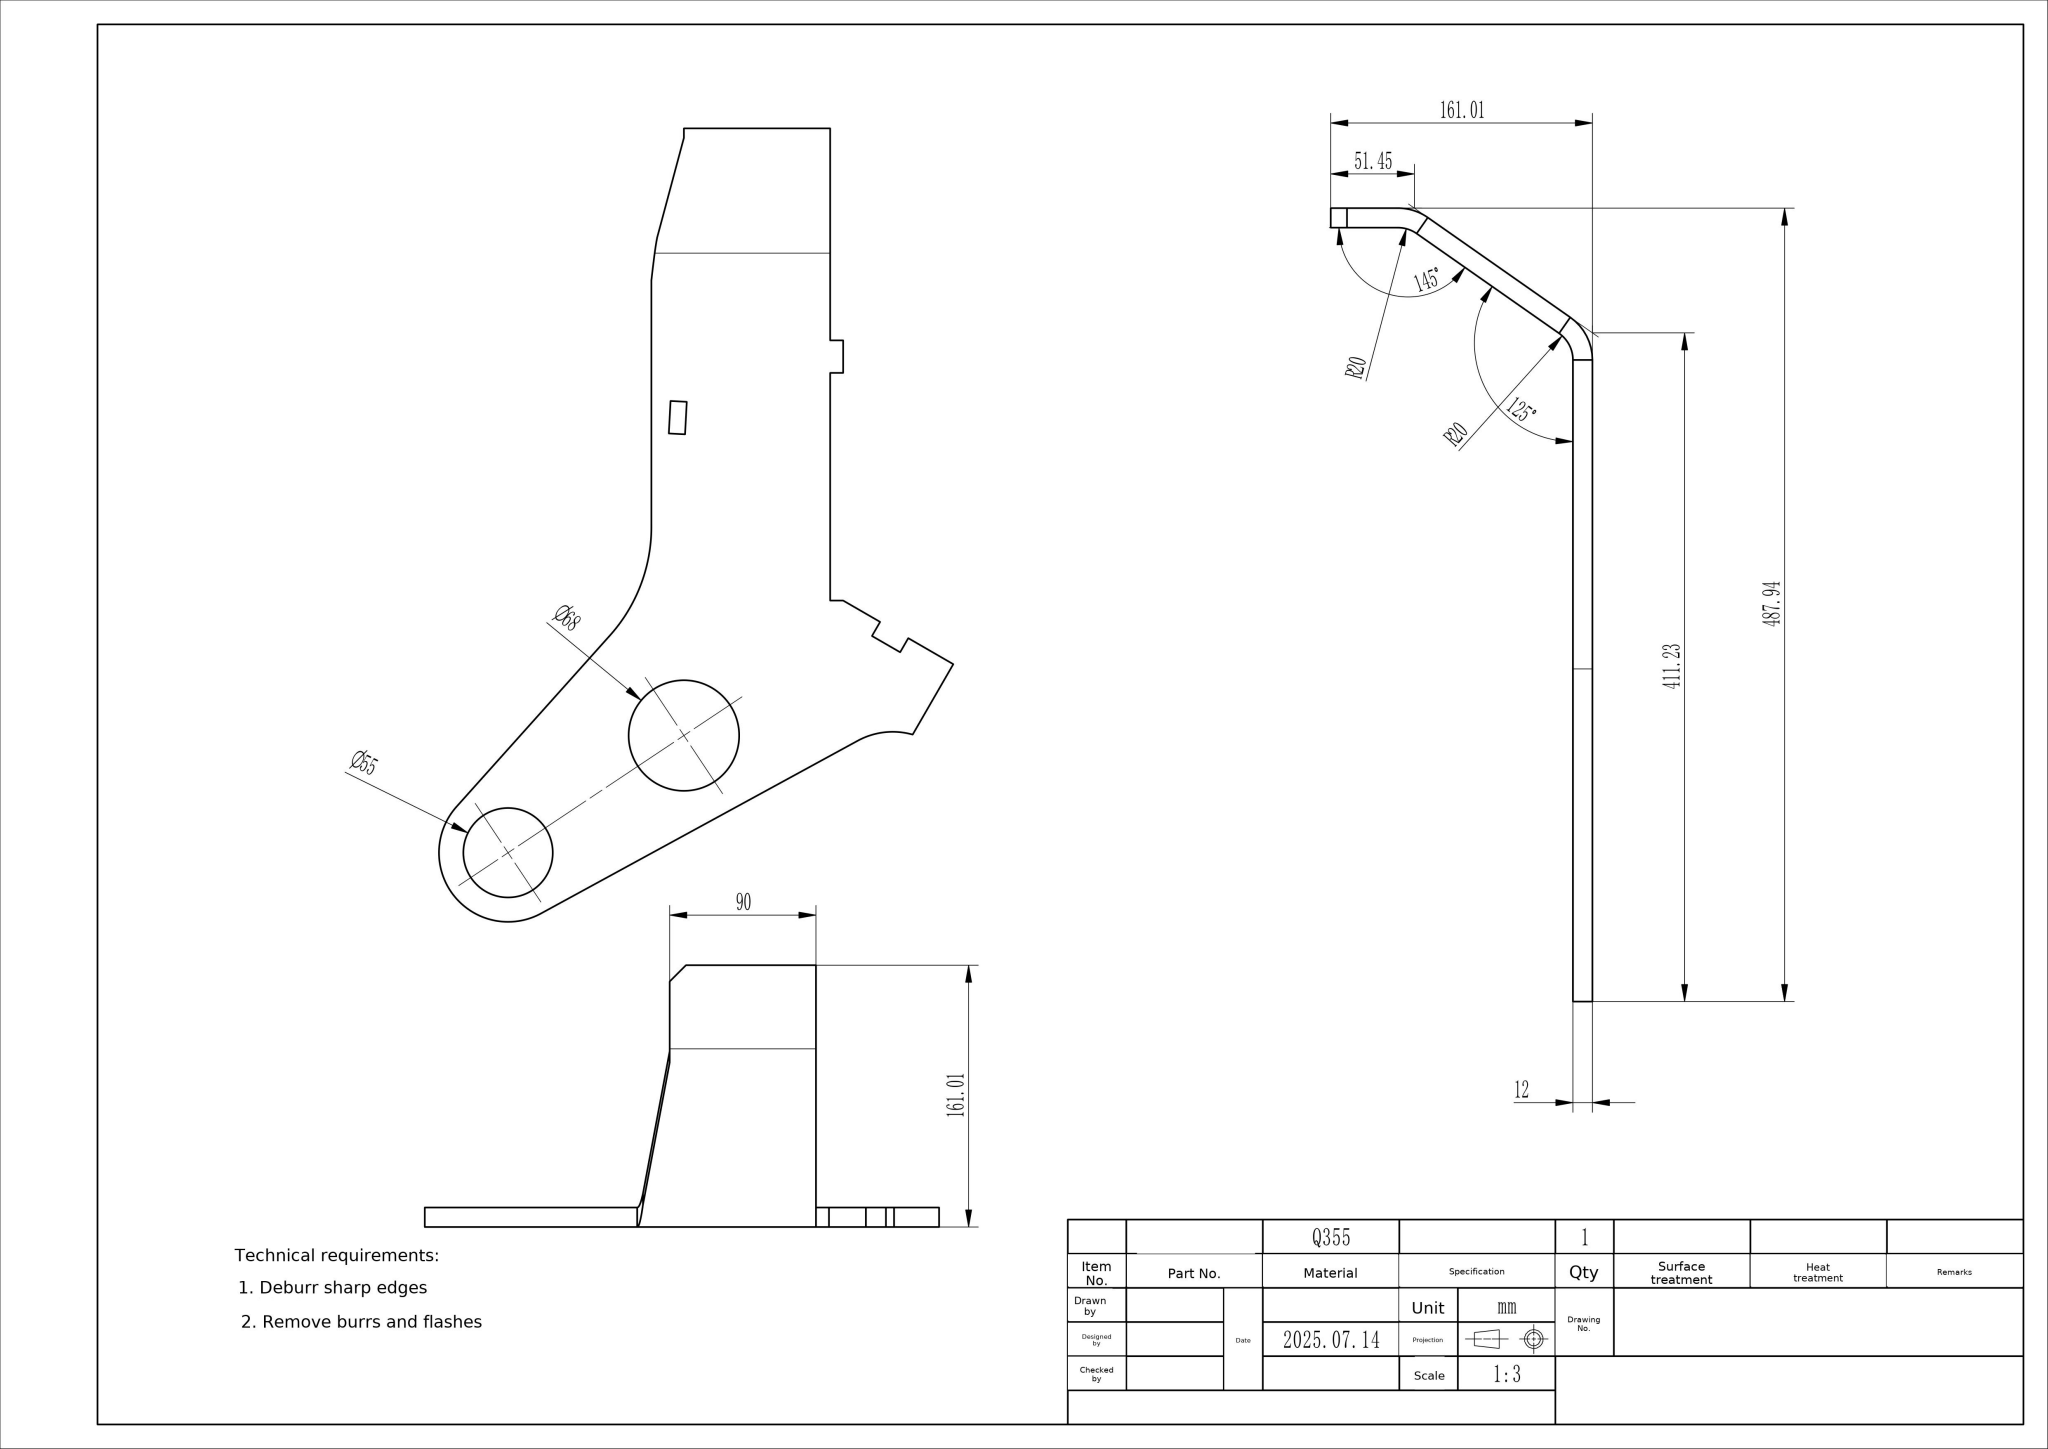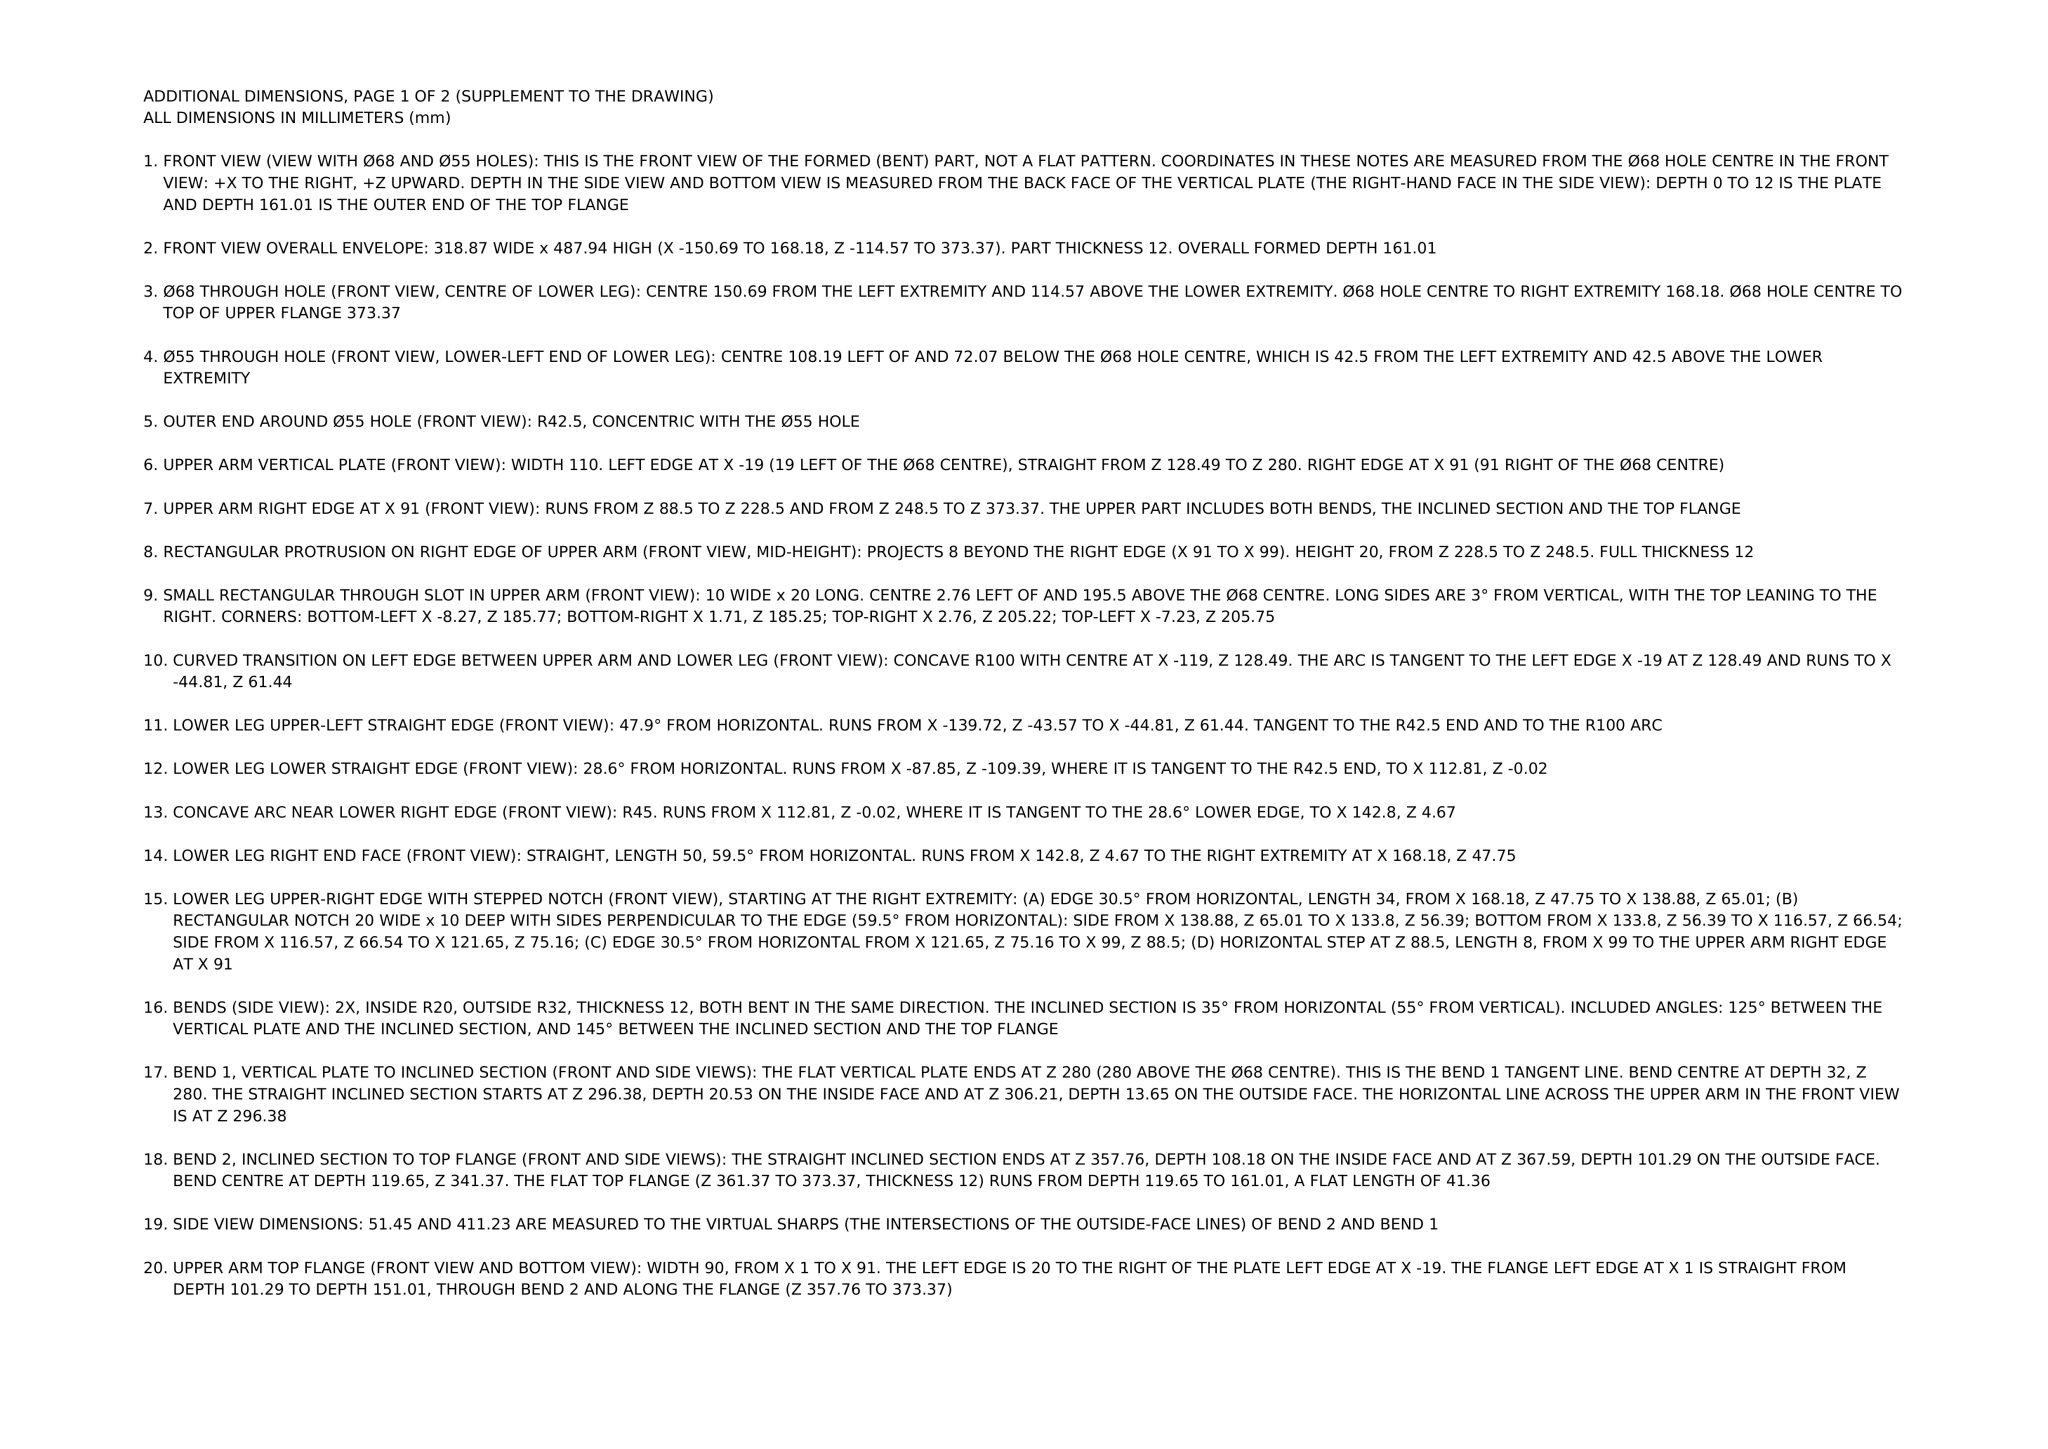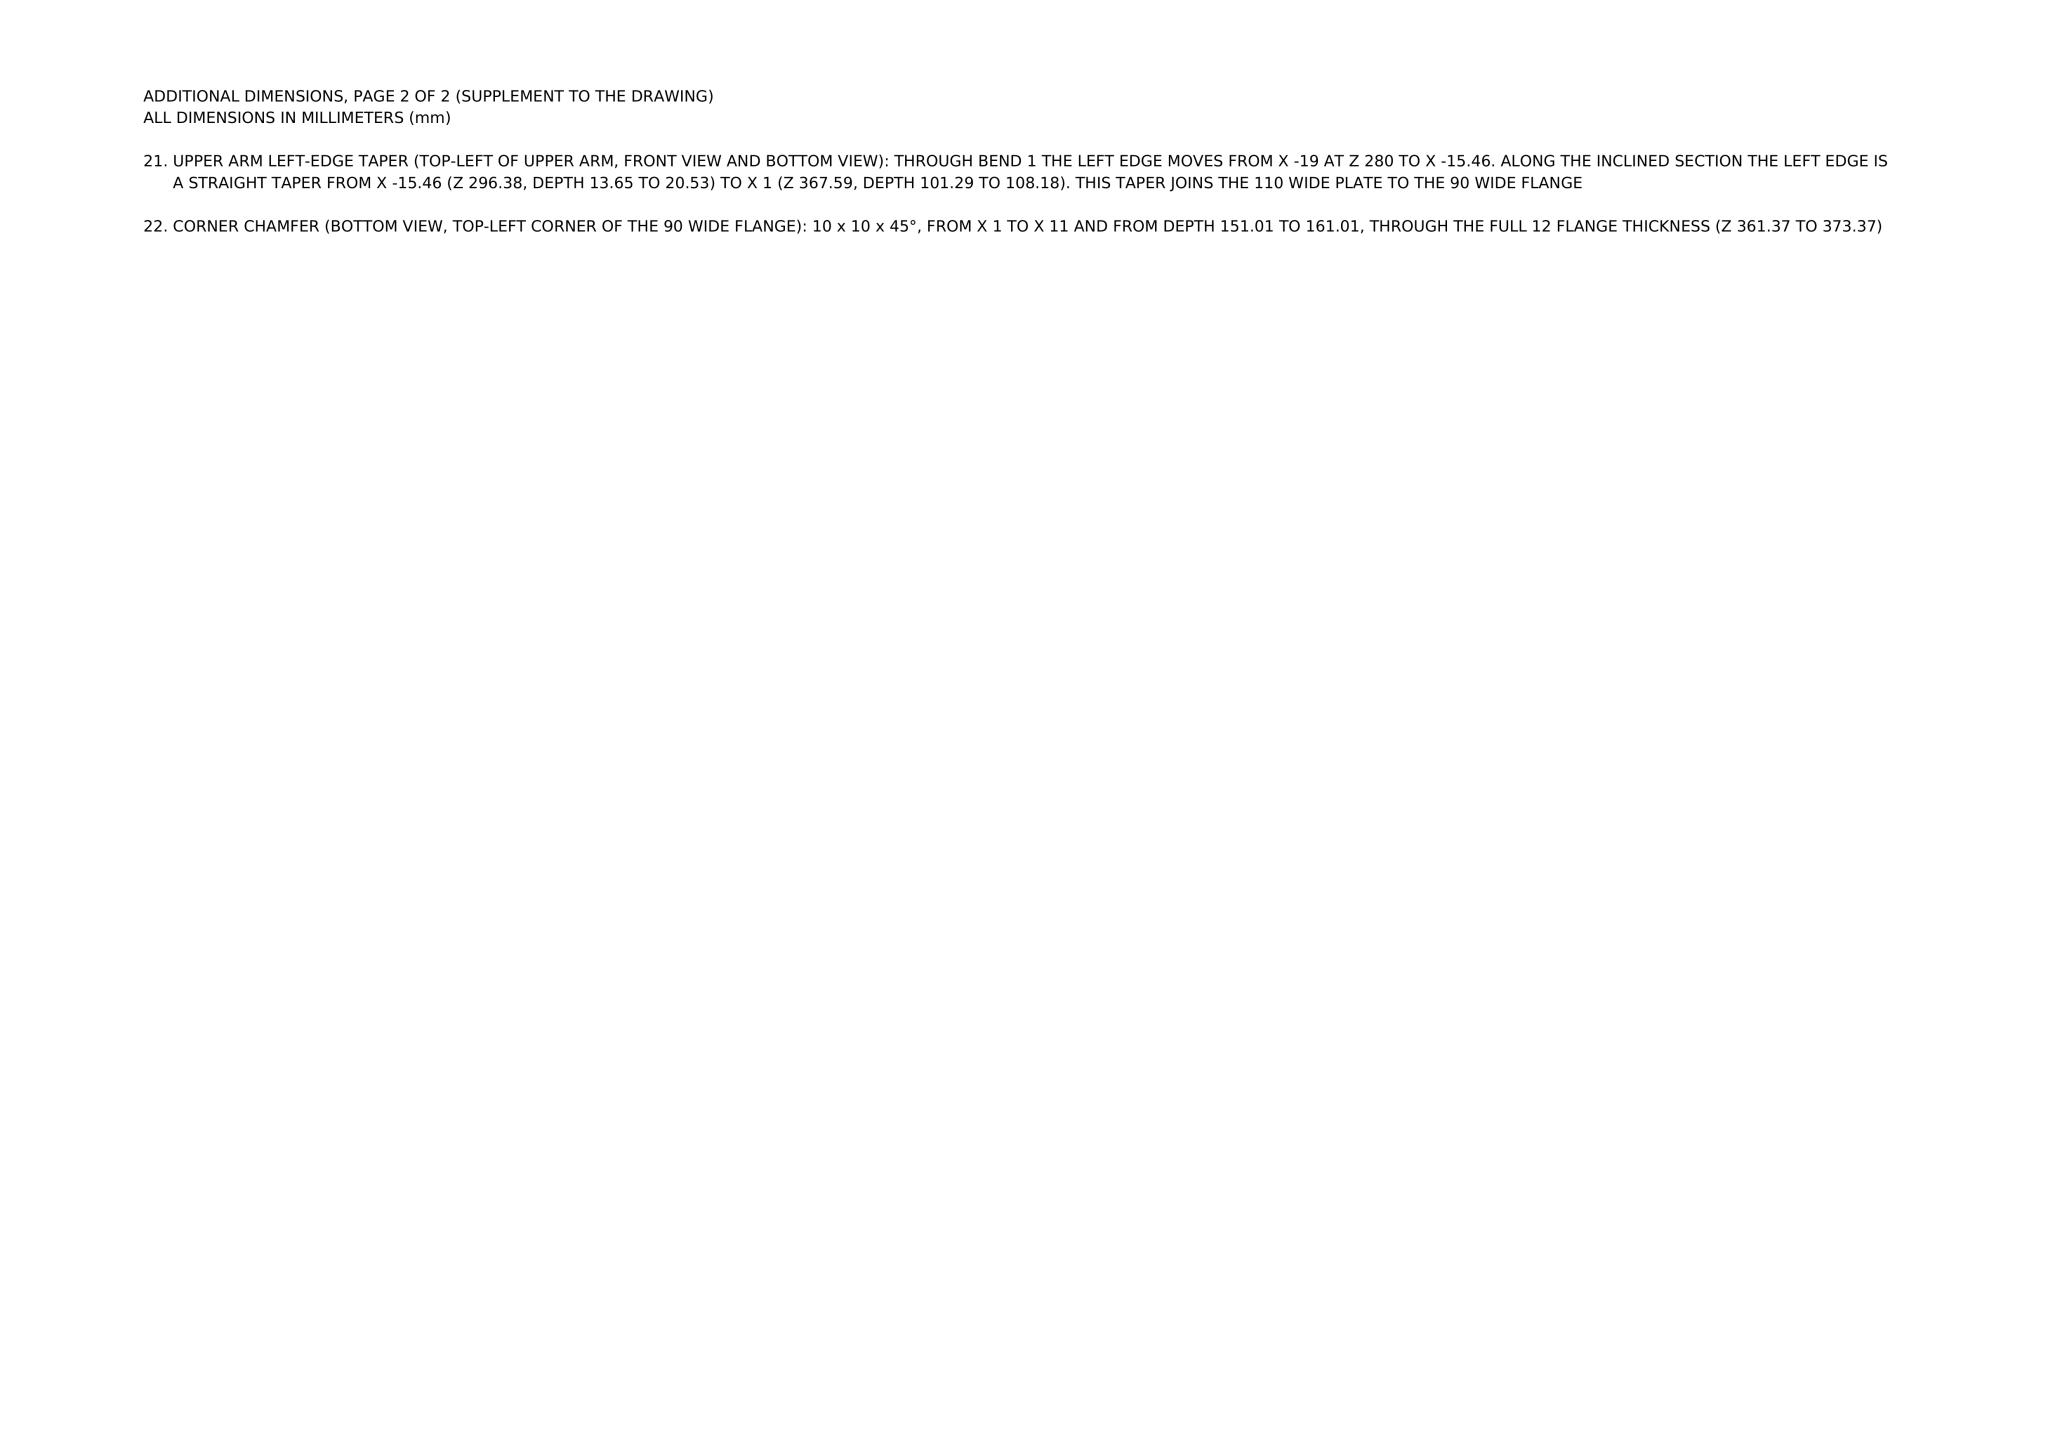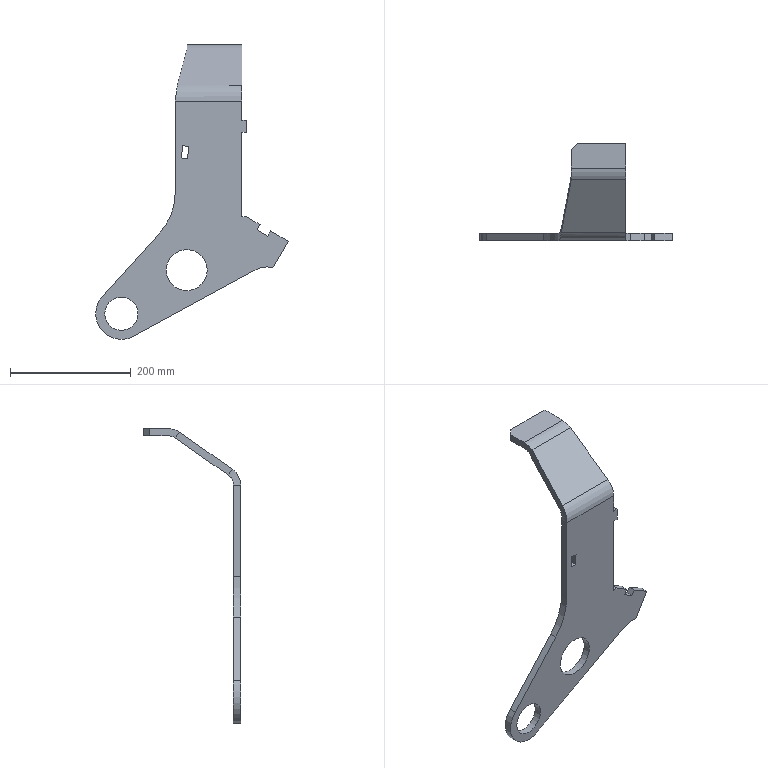Part | NX | mm | 1 solid | 39 faces | box 318.87 x 161.01 x 487.94 mm | volume 811844 mm3 | plane 29 | cylinder 9 | spline 1 | commonest cylinder face diameters 64 x2 40 x2 85 x1 90 x1 68 x1 55 x1 200 x1